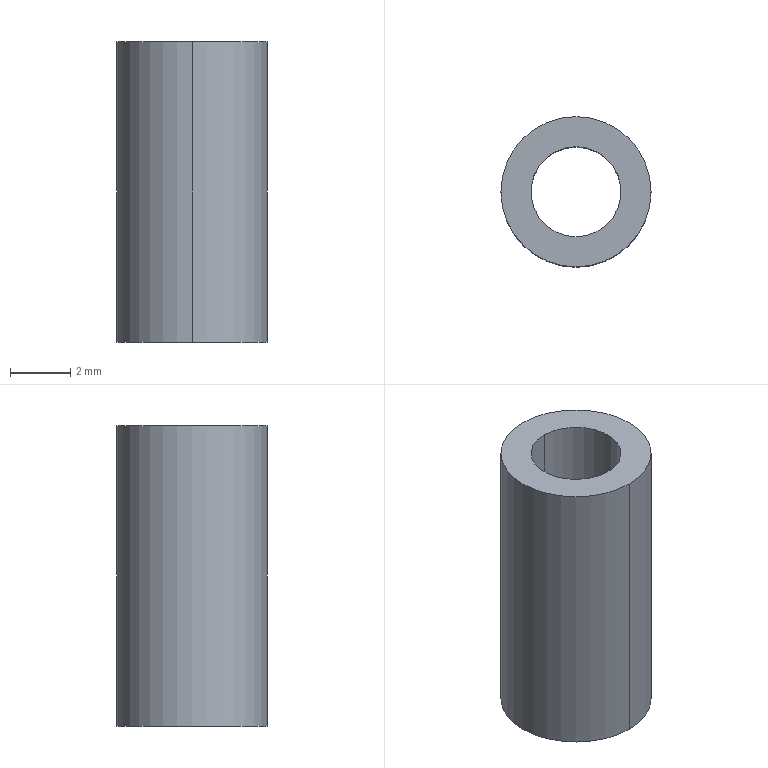Component | SolidWorks | Gimbal-1_10Pillar-3 | 1 solid | 6 faces | box 5 x 5 x 10 mm | volume 126 mm3 | cylinder 4 | plane 2 | commonest cylinder face diameters 3 x2 5 x2
build123d program:
from build123d import *

# Parameters (mm, degrees)
SKETCH1_R           = 2.5
SKETCH1_R_2         = 1.5
BOSS_EXTRUDE1_DEPTH = 10


with BuildPart() as part:
    # Sketch1 → Boss-Extrude1 (new body)
    with BuildSketch(Plane.XY):
        Circle(SKETCH1_R)
        Circle(SKETCH1_R_2, mode=Mode.SUBTRACT)
    extrude(amount=BOSS_EXTRUDE1_DEPTH)


solid = part.part

# Placed as in the assembly
solid = solid.moved(Location((26.5, 123, -31), (0, 0, 0)))
STEP:
#1=CARTESIAN_POINT('',(1.043,4.783,-1.22));
#2=VERTEX_POINT('',#1);
#3=CARTESIAN_POINT('',(1.043,4.902,-1.22));
#4=VERTEX_POINT('',#3);
#5=CARTESIAN_POINT('',(1.043,4.843,-1.22));
#6=DIRECTION('',(0.,0.,-1.));
#7=DIRECTION('',(-0.,1.,0.));
#8=AXIS2_PLACEMENT_3D('',#5,#6,#7);
#9=CIRCLE('',#8,0.05906);
#10=EDGE_CURVE('',#2,#4,#9,.T.);
#11=ORIENTED_EDGE('',*,*,#10,.T.);
#12=CARTESIAN_POINT('',(1.043,4.902,-0.8268));
#13=VERTEX_POINT('',#12);
#14=CARTESIAN_POINT('',(1.043,4.902,-1.22));
#15=DIRECTION('',(0.,0.,1.));
#16=VECTOR('',#15,39.37);
#17=LINE('',#14,#16);
#18=EDGE_CURVE('',#4,#13,#17,.T.);
#19=ORIENTED_EDGE('',*,*,#18,.T.);
#20=CARTESIAN_POINT('',(1.043,4.783,-0.8268));
#21=VERTEX_POINT('',#20);
#22=CARTESIAN_POINT('',(1.043,4.843,-0.8268));
#23=DIRECTION('',(0.,0.,-1.));
#24=DIRECTION('',(-0.,1.,0.));
#25=AXIS2_PLACEMENT_3D('',#22,#23,#24);
#26=CIRCLE('',#25,0.05906);
#27=EDGE_CURVE('',#21,#13,#26,.T.);
#28=ORIENTED_EDGE('',*,*,#27,.F.);
#29=CARTESIAN_POINT('',(1.043,4.783,-1.22));
#30=DIRECTION('',(0.,0.,1.));
#31=VECTOR('',#30,39.37);
#32=LINE('',#29,#31);
#33=EDGE_CURVE('',#2,#21,#32,.T.);
#34=ORIENTED_EDGE('',*,*,#33,.F.);
#35=EDGE_LOOP('',(#11,#19,#28,#34));
#36=FACE_OUTER_BOUND('',#35,.T.);
#37=CARTESIAN_POINT('',(1.043,4.843,-1.22));
#38=DIRECTION('',(0.,0.,1.));
#39=DIRECTION('',(0.,-1.,0.));
#40=AXIS2_PLACEMENT_3D('',#37,#38,#39);
#41=CYLINDRICAL_SURFACE('',#40,0.05906);
#42=ADVANCED_FACE('',(#36),#41,.F.);
#43=CARTESIAN_POINT('',(1.043,4.941,-1.22));
#44=VERTEX_POINT('',#43);
#45=CARTESIAN_POINT('',(1.043,4.744,-1.22));
#46=VERTEX_POINT('',#45);
#47=CARTESIAN_POINT('',(1.043,4.843,-1.22));
#48=DIRECTION('',(0.,0.,-1.));
#49=DIRECTION('',(-0.,1.,0.));
#50=AXIS2_PLACEMENT_3D('',#47,#48,#49);
#51=CIRCLE('',#50,0.09843);
#52=EDGE_CURVE('',#44,#46,#51,.T.);
#53=ORIENTED_EDGE('',*,*,#52,.F.);
#54=CARTESIAN_POINT('',(1.043,4.941,-0.8268));
#55=VERTEX_POINT('',#54);
#56=CARTESIAN_POINT('',(1.043,4.941,-1.22));
#57=DIRECTION('',(0.,0.,1.));
#58=VECTOR('',#57,39.37);
#59=LINE('',#56,#58);
#60=EDGE_CURVE('',#44,#55,#59,.T.);
#61=ORIENTED_EDGE('',*,*,#60,.T.);
#62=CARTESIAN_POINT('',(1.043,4.744,-0.8268));
#63=VERTEX_POINT('',#62);
#64=CARTESIAN_POINT('',(1.043,4.843,-0.8268));
#65=DIRECTION('',(0.,0.,-1.));
#66=DIRECTION('',(-0.,1.,0.));
#67=AXIS2_PLACEMENT_3D('',#64,#65,#66);
#68=CIRCLE('',#67,0.09843);
#69=EDGE_CURVE('',#55,#63,#68,.T.);
#70=ORIENTED_EDGE('',*,*,#69,.T.);
#71=CARTESIAN_POINT('',(1.043,4.744,-1.22));
#72=DIRECTION('',(0.,0.,1.));
#73=VECTOR('',#72,39.37);
#74=LINE('',#71,#73);
#75=EDGE_CURVE('',#46,#63,#74,.T.);
#76=ORIENTED_EDGE('',*,*,#75,.F.);
#77=EDGE_LOOP('',(#53,#61,#70,#76));
#78=FACE_OUTER_BOUND('',#77,.T.);
#79=CARTESIAN_POINT('',(1.043,4.843,-1.22));
#80=DIRECTION('',(0.,0.,1.));
#81=DIRECTION('',(0.,-1.,0.));
#82=AXIS2_PLACEMENT_3D('',#79,#80,#81);
#83=CYLINDRICAL_SURFACE('',#82,0.09843);
#84=ADVANCED_FACE('',(#78),#83,.T.);
#85=CARTESIAN_POINT('',(1.043,4.843,-1.22));
#86=DIRECTION('',(0.,0.,-1.));
#87=DIRECTION('',(-0.,1.,0.));
#88=AXIS2_PLACEMENT_3D('',#85,#86,#87);
#89=CIRCLE('',#88,0.09843);
#90=EDGE_CURVE('',#46,#44,#89,.T.);
#91=ORIENTED_EDGE('',*,*,#90,.T.);
#92=ORIENTED_EDGE('',*,*,#52,.T.);
#93=EDGE_LOOP('',(#91,#92));
#94=FACE_OUTER_BOUND('',#93,.T.);
#95=ORIENTED_EDGE('',*,*,#10,.F.);
#96=CARTESIAN_POINT('',(1.043,4.843,-1.22));
#97=DIRECTION('',(0.,0.,-1.));
#98=DIRECTION('',(-0.,1.,0.));
#99=AXIS2_PLACEMENT_3D('',#96,#97,#98);
#100=CIRCLE('',#99,0.05906);
#101=EDGE_CURVE('',#4,#2,#100,.T.);
#102=ORIENTED_EDGE('',*,*,#101,.F.);
#103=EDGE_LOOP('',(#95,#102));
#104=FACE_BOUND('',#103,.T.);
#105=CARTESIAN_POINT('',(1.043,4.843,-1.22));
#106=DIRECTION('',(0.,0.,-1.));
#107=DIRECTION('',(-0.,1.,0.));
#108=AXIS2_PLACEMENT_3D('',#105,#106,#107);
#109=PLANE('',#108);
#110=ADVANCED_FACE('',(#94,#104),#109,.T.);
#111=CARTESIAN_POINT('',(1.043,4.843,-0.8268));
#112=DIRECTION('',(0.,0.,-1.));
#113=DIRECTION('',(-0.,1.,0.));
#114=AXIS2_PLACEMENT_3D('',#111,#112,#113);
#115=CIRCLE('',#114,0.09843);
#116=EDGE_CURVE('',#63,#55,#115,.T.);
#117=ORIENTED_EDGE('',*,*,#116,.F.);
#118=ORIENTED_EDGE('',*,*,#69,.F.);
#119=EDGE_LOOP('',(#117,#118));
#120=FACE_OUTER_BOUND('',#119,.T.);
#121=ORIENTED_EDGE('',*,*,#27,.T.);
#122=CARTESIAN_POINT('',(1.043,4.843,-0.8268));
#123=DIRECTION('',(0.,0.,-1.));
#124=DIRECTION('',(-0.,1.,0.));
#125=AXIS2_PLACEMENT_3D('',#122,#123,#124);
#126=CIRCLE('',#125,0.05906);
#127=EDGE_CURVE('',#13,#21,#126,.T.);
#128=ORIENTED_EDGE('',*,*,#127,.T.);
#129=EDGE_LOOP('',(#121,#128));
#130=FACE_BOUND('',#129,.T.);
#131=CARTESIAN_POINT('',(1.043,4.843,-0.8268));
#132=DIRECTION('',(0.,0.,-1.));
#133=DIRECTION('',(-0.,1.,0.));
#134=AXIS2_PLACEMENT_3D('',#131,#132,#133);
#135=PLANE('',#134);
#136=ADVANCED_FACE('',(#120,#130),#135,.F.);
#137=ORIENTED_EDGE('',*,*,#60,.F.);
#138=ORIENTED_EDGE('',*,*,#90,.F.);
#139=ORIENTED_EDGE('',*,*,#75,.T.);
#140=ORIENTED_EDGE('',*,*,#116,.T.);
#141=EDGE_LOOP('',(#137,#138,#139,#140));
#142=FACE_OUTER_BOUND('',#141,.T.);
#143=CARTESIAN_POINT('',(1.043,4.843,-1.22));
#144=DIRECTION('',(0.,0.,1.));
#145=DIRECTION('',(0.,-1.,0.));
#146=AXIS2_PLACEMENT_3D('',#143,#144,#145);
#147=CYLINDRICAL_SURFACE('',#146,0.09843);
#148=ADVANCED_FACE('',(#142),#147,.T.);
#149=ORIENTED_EDGE('',*,*,#18,.F.);
#150=ORIENTED_EDGE('',*,*,#101,.T.);
#151=ORIENTED_EDGE('',*,*,#33,.T.);
#152=ORIENTED_EDGE('',*,*,#127,.F.);
#153=EDGE_LOOP('',(#149,#150,#151,#152));
#154=FACE_OUTER_BOUND('',#153,.T.);
#155=CARTESIAN_POINT('',(1.043,4.843,-1.22));
#156=DIRECTION('',(0.,0.,1.));
#157=DIRECTION('',(0.,-1.,0.));
#158=AXIS2_PLACEMENT_3D('',#155,#156,#157);
#159=CYLINDRICAL_SURFACE('',#158,0.05906);
#160=ADVANCED_FACE('',(#154),#159,.F.);
#161=CLOSED_SHELL('',(#42,#84,#110,#136,#148,#160));
#162=MANIFOLD_SOLID_BREP('',#161);
#163=CARTESIAN_POINT('',(0.,0.,0.));
#164=DIRECTION('',(0.,0.,1.));
#165=DIRECTION('',(1.,0.,0.));
#166=AXIS2_PLACEMENT_3D('',#163,#164,#165);
#167=(LENGTH_UNIT()NAMED_UNIT(*)SI_UNIT($,.METRE.));
#168=LENGTH_MEASURE_WITH_UNIT(LENGTH_MEASURE(0.0254),#167);
#169=DIMENSIONAL_EXPONENTS(1.,0.,0.,0.,0.,0.,0.);
#170=(CONVERSION_BASED_UNIT('',#168)LENGTH_UNIT()NAMED_UNIT(#169));
#171=UNCERTAINTY_MEASURE_WITH_UNIT(LENGTH_MEASURE(0.00001),#170,'','');
#172=(NAMED_UNIT(*)PLANE_ANGLE_UNIT()SI_UNIT($,.RADIAN.));
#173=(NAMED_UNIT(*)SI_UNIT($,.STERADIAN.)SOLID_ANGLE_UNIT());
#174=(GEOMETRIC_REPRESENTATION_CONTEXT(3)GLOBAL_UNCERTAINTY_ASSIGNED_CONTEXT((#171))GLOBAL_UNIT_ASSIGNED_CONTEXT((#170,#172,#173))REPRESENTATION_CONTEXT('',''));
#175=ADVANCED_BREP_SHAPE_REPRESENTATION('',(#162,#166),#174);
#176=COLOUR_RGB('',0.7922,0.8196,0.9333);
#177=FILL_AREA_STYLE_COLOUR('',#176);
#178=FILL_AREA_STYLE('',(#177));
#179=SURFACE_STYLE_FILL_AREA(#178);
#180=SURFACE_SIDE_STYLE('',(#179));
#181=SURFACE_STYLE_USAGE(.BOTH.,#180);
#182=PRESENTATION_STYLE_ASSIGNMENT((#181));
#183=STYLED_ITEM('',(#182),#162);
#184=PRESENTATION_LAYER_ASSIGNMENT('','',(#183));
#185=(LENGTH_UNIT()NAMED_UNIT(*)SI_UNIT($,.METRE.));
#186=LENGTH_MEASURE_WITH_UNIT(LENGTH_MEASURE(0.0254),#185);
#187=DIMENSIONAL_EXPONENTS(1.,0.,0.,0.,0.,0.,0.);
#188=(CONVERSION_BASED_UNIT('',#186)LENGTH_UNIT()NAMED_UNIT(#187));
#189=UNCERTAINTY_MEASURE_WITH_UNIT(LENGTH_MEASURE(0.00001),#188,'','');
#190=(NAMED_UNIT(*)PLANE_ANGLE_UNIT()SI_UNIT($,.RADIAN.));
#191=(NAMED_UNIT(*)SI_UNIT($,.STERADIAN.)SOLID_ANGLE_UNIT());
#192=(GEOMETRIC_REPRESENTATION_CONTEXT(3)GLOBAL_UNCERTAINTY_ASSIGNED_CONTEXT((#189))GLOBAL_UNIT_ASSIGNED_CONTEXT((#188,#190,#191))REPRESENTATION_CONTEXT('',''));
#193=MECHANICAL_DESIGN_GEOMETRIC_PRESENTATION_REPRESENTATION('',(#183),#192);